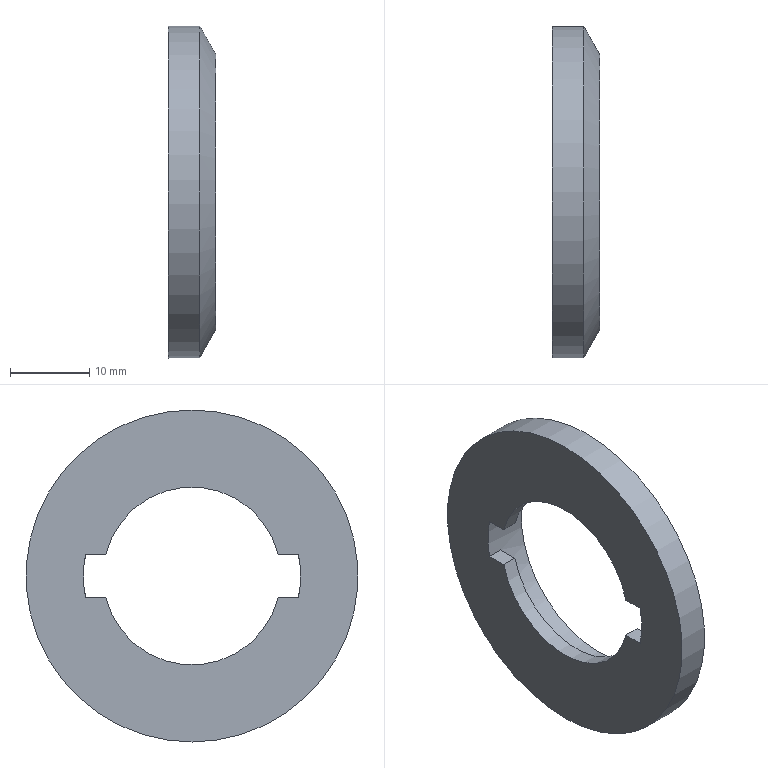Component | NX | SPACER_BLOCK | 1 solid | 13 faces | box 6 x 42 x 42 mm | volume 4639 mm3 | plane 8 | cylinder 4 | cone 1 | commonest cylinder face diameters 22.5 x2 42 x1 27.5 x1
STEP:
#1=CARTESIAN_POINT('',(0.,0.,0.));
#2=DIRECTION('',(0.,0.,1.));
#3=DIRECTION('',(1.,0.,0.));
#4=AXIS2_PLACEMENT_3D('',#1,#2,#3);
#5=CARTESIAN_POINT('',(-2.738,-11.881,-14.373));
#6=VERTEX_POINT('',#5);
#7=CARTESIAN_POINT('',(-2.738,-9.319,-14.373));
#8=VERTEX_POINT('',#7);
#9=CARTESIAN_POINT('',(-2.738,-11.881,-14.373));
#10=DIRECTION('',(0.,1.,0.));
#11=VECTOR('',#10,1.);
#12=LINE('',#9,#11);
#13=CARTESIAN_POINT('',(-2.738,1.601,-11.667));
#14=DIRECTION('',(-1.,0.,0.));
#15=DIRECTION('',(0.,0.,1.));
#16=AXIS2_PLACEMENT_3D('',#13,#14,#15);
#17=PLANE('',#16);
#18=CARTESIAN_POINT('',(-2.706,-13.481));
#19=DIRECTION('',(0.,1.));
#20=VECTOR('',#19,1.);
#21=LINE('',#18,#20);
#22=(GEOMETRIC_REPRESENTATION_CONTEXT(2)PARAMETRIC_REPRESENTATION_CONTEXT()REPRESENTATION_CONTEXT('',''));
#23=DEFINITIONAL_REPRESENTATION('',(#21),#22);
#24=PCURVE('',#17,#23);
#25=CARTESIAN_POINT('',(-12.738,-11.881,-14.373));
#26=DIRECTION('',(0.,0.,-1.));
#27=DIRECTION('',(0.,1.,0.));
#28=AXIS2_PLACEMENT_3D('',#25,#26,#27);
#29=PLANE('',#28);
#30=CARTESIAN_POINT('',(0.,10.));
#31=DIRECTION('',(1.,0.));
#32=VECTOR('',#31,1.);
#33=LINE('',#30,#32);
#34=(GEOMETRIC_REPRESENTATION_CONTEXT(2)PARAMETRIC_REPRESENTATION_CONTEXT()REPRESENTATION_CONTEXT('',''));
#35=DEFINITIONAL_REPRESENTATION('',(#33),#34);
#36=PCURVE('',#29,#35);
#37=SURFACE_CURVE('',#12,(#24,#36),.PCURVE_S1.);
#38=EDGE_CURVE('',#6,#8,#37,.T.);
#39=ORIENTED_EDGE('',*,*,#38,.F.);
#40=CARTESIAN_POINT('',(-2.738,1.601,-25.417));
#41=VERTEX_POINT('',#40);
#42=CARTESIAN_POINT('',(-2.738,1.601,-11.667));
#43=DIRECTION('',(-1.,0.,0.));
#44=DIRECTION('',(0.,0.,-1.));
#45=AXIS2_PLACEMENT_3D('',#42,#43,#44);
#46=CIRCLE('',#45,13.75);
#47=CARTESIAN_POINT('',(0.,0.));
#48=DIRECTION('',(-1.,0.));
#49=AXIS2_PLACEMENT_2D('',#47,#48);
#50=CIRCLE('',#49,13.75);
#51=(GEOMETRIC_REPRESENTATION_CONTEXT(2)PARAMETRIC_REPRESENTATION_CONTEXT()REPRESENTATION_CONTEXT('',''));
#52=DEFINITIONAL_REPRESENTATION('',(#50),#51);
#53=PCURVE('',#17,#52);
#54=CARTESIAN_POINT('',(1.262,1.601,-11.667));
#55=DIRECTION('',(-1.,0.,0.));
#56=DIRECTION('',(0.,0.,-1.));
#57=AXIS2_PLACEMENT_3D('',#54,#55,#56);
#58=CYLINDRICAL_SURFACE('',#57,13.75);
#59=CARTESIAN_POINT('',(-6.283,4.));
#60=DIRECTION('',(1.,0.));
#61=VECTOR('',#60,1.);
#62=LINE('',#59,#61);
#63=(GEOMETRIC_REPRESENTATION_CONTEXT(2)PARAMETRIC_REPRESENTATION_CONTEXT()REPRESENTATION_CONTEXT('',''));
#64=DEFINITIONAL_REPRESENTATION('',(#62),#63);
#65=PCURVE('',#58,#64);
#66=SURFACE_CURVE('',#46,(#53,#65),.PCURVE_S1.);
#67=EDGE_CURVE('',#41,#6,#66,.T.);
#68=ORIENTED_EDGE('',*,*,#67,.F.);
#69=CARTESIAN_POINT('',(-2.738,15.082,-14.373));
#70=VERTEX_POINT('',#69);
#71=CARTESIAN_POINT('',(-2.738,1.601,-11.667));
#72=DIRECTION('',(-1.,0.,0.));
#73=DIRECTION('',(0.,0.,-1.));
#74=AXIS2_PLACEMENT_3D('',#71,#72,#73);
#75=CIRCLE('',#74,13.75);
#76=CARTESIAN_POINT('',(0.,0.));
#77=DIRECTION('',(-1.,0.));
#78=AXIS2_PLACEMENT_2D('',#76,#77);
#79=CIRCLE('',#78,13.75);
#80=(GEOMETRIC_REPRESENTATION_CONTEXT(2)PARAMETRIC_REPRESENTATION_CONTEXT()REPRESENTATION_CONTEXT('',''));
#81=DEFINITIONAL_REPRESENTATION('',(#79),#80);
#82=PCURVE('',#17,#81);
#83=CARTESIAN_POINT('',(0.,4.));
#84=DIRECTION('',(1.,0.));
#85=VECTOR('',#84,1.);
#86=LINE('',#83,#85);
#87=(GEOMETRIC_REPRESENTATION_CONTEXT(2)PARAMETRIC_REPRESENTATION_CONTEXT()REPRESENTATION_CONTEXT('',''));
#88=DEFINITIONAL_REPRESENTATION('',(#86),#87);
#89=PCURVE('',#58,#88);
#90=SURFACE_CURVE('',#75,(#82,#89),.PCURVE_S1.);
#91=EDGE_CURVE('',#70,#41,#90,.T.);
#92=ORIENTED_EDGE('',*,*,#91,.F.);
#93=CARTESIAN_POINT('',(-2.738,12.52,-14.373));
#94=VERTEX_POINT('',#93);
#95=CARTESIAN_POINT('',(-2.738,12.52,-14.373));
#96=DIRECTION('',(0.,1.,0.));
#97=VECTOR('',#96,1.);
#98=LINE('',#95,#97);
#99=CARTESIAN_POINT('',(-2.706,10.92));
#100=DIRECTION('',(0.,1.));
#101=VECTOR('',#100,1.);
#102=LINE('',#99,#101);
#103=(GEOMETRIC_REPRESENTATION_CONTEXT(2)PARAMETRIC_REPRESENTATION_CONTEXT()REPRESENTATION_CONTEXT('',''));
#104=DEFINITIONAL_REPRESENTATION('',(#102),#103);
#105=PCURVE('',#17,#104);
#106=CARTESIAN_POINT('',(-12.738,12.52,-14.373));
#107=DIRECTION('',(0.,0.,-1.));
#108=DIRECTION('',(0.,1.,0.));
#109=AXIS2_PLACEMENT_3D('',#106,#107,#108);
#110=PLANE('',#109);
#111=CARTESIAN_POINT('',(0.,10.));
#112=DIRECTION('',(1.,0.));
#113=VECTOR('',#112,1.);
#114=LINE('',#111,#113);
#115=(GEOMETRIC_REPRESENTATION_CONTEXT(2)PARAMETRIC_REPRESENTATION_CONTEXT()REPRESENTATION_CONTEXT('',''));
#116=DEFINITIONAL_REPRESENTATION('',(#114),#115);
#117=PCURVE('',#110,#116);
#118=SURFACE_CURVE('',#98,(#105,#117),.PCURVE_S1.);
#119=EDGE_CURVE('',#94,#70,#118,.T.);
#120=ORIENTED_EDGE('',*,*,#119,.F.);
#121=CARTESIAN_POINT('',(-2.738,1.601,-11.667));
#122=DIRECTION('',(1.,0.,0.));
#123=DIRECTION('',(0.,0.,-1.));
#124=AXIS2_PLACEMENT_3D('',#121,#122,#123);
#125=CIRCLE('',#124,11.25);
#126=CARTESIAN_POINT('',(-11.25,0.));
#127=CARTESIAN_POINT('',(-11.25,19.486));
#128=CARTESIAN_POINT('',(5.625,9.743));
#129=CARTESIAN_POINT('',(22.5,0.));
#130=CARTESIAN_POINT('',(5.625,-9.743));
#131=CARTESIAN_POINT('',(-11.25,-19.486));
#132=CARTESIAN_POINT('',(-11.25,0.));
#133=(BOUNDED_CURVE()B_SPLINE_CURVE(2,(#126,#127,#128,#129,#130,#131,#132),.UNSPECIFIED.,.T.,.F.)B_SPLINE_CURVE_WITH_KNOTS((1,2,2,2,2,1),(-2.094,0.,2.094,4.189,6.283,8.378),.UNSPECIFIED.)CURVE()GEOMETRIC_REPRESENTATION_ITEM()RATIONAL_B_SPLINE_CURVE((1.,0.5,1.,0.5,1.,0.5,1.))REPRESENTATION_ITEM(''));
#134=(GEOMETRIC_REPRESENTATION_CONTEXT(2)PARAMETRIC_REPRESENTATION_CONTEXT()REPRESENTATION_CONTEXT('',''));
#135=DEFINITIONAL_REPRESENTATION('',(#133),#134);
#136=PCURVE('',#17,#135);
#137=CARTESIAN_POINT('',(-12.738,1.601,-11.667));
#138=DIRECTION('',(1.,0.,0.));
#139=DIRECTION('',(0.,0.,-1.));
#140=AXIS2_PLACEMENT_3D('',#137,#138,#139);
#141=CYLINDRICAL_SURFACE('',#140,11.25);
#142=CARTESIAN_POINT('',(0.,10.));
#143=DIRECTION('',(1.,0.));
#144=VECTOR('',#143,1.);
#145=LINE('',#142,#144);
#146=(GEOMETRIC_REPRESENTATION_CONTEXT(2)PARAMETRIC_REPRESENTATION_CONTEXT()REPRESENTATION_CONTEXT('',''));
#147=DEFINITIONAL_REPRESENTATION('',(#145),#146);
#148=PCURVE('',#141,#147);
#149=SURFACE_CURVE('',#125,(#136,#148),.PCURVE_S1.);
#150=EDGE_CURVE('',#8,#94,#149,.T.);
#151=ORIENTED_EDGE('',*,*,#150,.F.);
#152=EDGE_LOOP('',(#39,#68,#92,#120,#151));
#153=FACE_BOUND('',#152,.T.);
#154=ADVANCED_FACE('',(#153),#17,.F.);
#155=CARTESIAN_POINT('',(-4.738,-11.881,-8.961));
#156=VERTEX_POINT('',#155);
#157=CARTESIAN_POINT('',(-4.738,-9.319,-8.961));
#158=VERTEX_POINT('',#157);
#159=CARTESIAN_POINT('',(-4.738,-19.399,-8.961));
#160=DIRECTION('',(0.,1.,0.));
#161=VECTOR('',#160,1.);
#162=LINE('',#159,#161);
#163=CARTESIAN_POINT('',(-4.738,-19.399,-11.667));
#164=DIRECTION('',(-1.,0.,0.));
#165=DIRECTION('',(0.,0.,1.));
#166=AXIS2_PLACEMENT_3D('',#163,#164,#165);
#167=PLANE('',#166);
#168=CARTESIAN_POINT('',(2.706,0.));
#169=DIRECTION('',(0.,1.));
#170=VECTOR('',#169,1.);
#171=LINE('',#168,#170);
#172=(GEOMETRIC_REPRESENTATION_CONTEXT(2)PARAMETRIC_REPRESENTATION_CONTEXT()REPRESENTATION_CONTEXT('',''));
#173=DEFINITIONAL_REPRESENTATION('',(#171),#172);
#174=PCURVE('',#167,#173);
#175=CARTESIAN_POINT('',(-12.738,-9.319,-8.961));
#176=DIRECTION('',(0.,-0.,1.));
#177=DIRECTION('',(0.,-1.,-0.));
#178=AXIS2_PLACEMENT_3D('',#175,#176,#177);
#179=PLANE('',#178);
#180=CARTESIAN_POINT('',(10.08,8.));
#181=DIRECTION('',(-1.,0.));
#182=VECTOR('',#181,1.);
#183=LINE('',#180,#182);
#184=(GEOMETRIC_REPRESENTATION_CONTEXT(2)PARAMETRIC_REPRESENTATION_CONTEXT()REPRESENTATION_CONTEXT('',''));
#185=DEFINITIONAL_REPRESENTATION('',(#183),#184);
#186=PCURVE('',#179,#185);
#187=SURFACE_CURVE('',#162,(#174,#186),.PCURVE_S1.);
#188=EDGE_CURVE('',#156,#158,#187,.T.);
#189=ORIENTED_EDGE('',*,*,#188,.F.);
#190=CARTESIAN_POINT('',(-4.738,-11.881,-14.373));
#191=VERTEX_POINT('',#190);
#192=CARTESIAN_POINT('',(-4.738,1.601,-11.667));
#193=DIRECTION('',(-1.,0.,0.));
#194=DIRECTION('',(0.,0.,1.));
#195=AXIS2_PLACEMENT_3D('',#192,#193,#194);
#196=CIRCLE('',#195,13.75);
#197=CARTESIAN_POINT('',(0.,21.));
#198=DIRECTION('',(1.,0.));
#199=AXIS2_PLACEMENT_2D('',#197,#198);
#200=CIRCLE('',#199,13.75);
#201=(GEOMETRIC_REPRESENTATION_CONTEXT(2)PARAMETRIC_REPRESENTATION_CONTEXT()REPRESENTATION_CONTEXT('',''));
#202=DEFINITIONAL_REPRESENTATION('',(#200),#201);
#203=PCURVE('',#167,#202);
#204=CARTESIAN_POINT('',(-3.142,6.));
#205=DIRECTION('',(1.,0.));
#206=VECTOR('',#205,1.);
#207=LINE('',#204,#206);
#208=(GEOMETRIC_REPRESENTATION_CONTEXT(2)PARAMETRIC_REPRESENTATION_CONTEXT()REPRESENTATION_CONTEXT('',''));
#209=DEFINITIONAL_REPRESENTATION('',(#207),#208);
#210=PCURVE('',#58,#209);
#211=SURFACE_CURVE('',#196,(#203,#210),.PCURVE_S1.);
#212=EDGE_CURVE('',#191,#156,#211,.T.);
#213=ORIENTED_EDGE('',*,*,#212,.F.);
#214=CARTESIAN_POINT('',(-4.738,-9.319,-14.373));
#215=VERTEX_POINT('',#214);
#216=CARTESIAN_POINT('',(-4.738,-19.399,-14.373));
#217=DIRECTION('',(0.,-1.,-0.));
#218=VECTOR('',#217,1.);
#219=LINE('',#216,#218);
#220=CARTESIAN_POINT('',(-2.706,0.));
#221=DIRECTION('',(-0.,-1.));
#222=VECTOR('',#221,1.);
#223=LINE('',#220,#222);
#224=(GEOMETRIC_REPRESENTATION_CONTEXT(2)PARAMETRIC_REPRESENTATION_CONTEXT()REPRESENTATION_CONTEXT('',''));
#225=DEFINITIONAL_REPRESENTATION('',(#223),#224);
#226=PCURVE('',#167,#225);
#227=CARTESIAN_POINT('',(-7.519,8.));
#228=DIRECTION('',(-1.,0.));
#229=VECTOR('',#228,1.);
#230=LINE('',#227,#229);
#231=(GEOMETRIC_REPRESENTATION_CONTEXT(2)PARAMETRIC_REPRESENTATION_CONTEXT()REPRESENTATION_CONTEXT('',''));
#232=DEFINITIONAL_REPRESENTATION('',(#230),#231);
#233=PCURVE('',#29,#232);
#234=SURFACE_CURVE('',#219,(#226,#233),.PCURVE_S1.);
#235=EDGE_CURVE('',#215,#191,#234,.T.);
#236=ORIENTED_EDGE('',*,*,#235,.F.);
#237=CARTESIAN_POINT('',(-4.738,12.52,-14.373));
#238=VERTEX_POINT('',#237);
#239=CARTESIAN_POINT('',(-4.738,1.601,-11.667));
#240=DIRECTION('',(-1.,0.,0.));
#241=DIRECTION('',(0.,0.,1.));
#242=AXIS2_PLACEMENT_3D('',#239,#240,#241);
#243=CIRCLE('',#242,11.25);
#244=CARTESIAN_POINT('',(0.,21.));
#245=DIRECTION('',(1.,0.));
#246=AXIS2_PLACEMENT_2D('',#244,#245);
#247=CIRCLE('',#246,11.25);
#248=(GEOMETRIC_REPRESENTATION_CONTEXT(2)PARAMETRIC_REPRESENTATION_CONTEXT()REPRESENTATION_CONTEXT('',''));
#249=DEFINITIONAL_REPRESENTATION('',(#247),#248);
#250=PCURVE('',#167,#249);
#251=CARTESIAN_POINT('',(9.425,8.));
#252=DIRECTION('',(-1.,0.));
#253=VECTOR('',#252,1.);
#254=LINE('',#251,#253);
#255=(GEOMETRIC_REPRESENTATION_CONTEXT(2)PARAMETRIC_REPRESENTATION_CONTEXT()REPRESENTATION_CONTEXT('',''));
#256=DEFINITIONAL_REPRESENTATION('',(#254),#255);
#257=PCURVE('',#141,#256);
#258=SURFACE_CURVE('',#243,(#250,#257),.PCURVE_S1.);
#259=EDGE_CURVE('',#238,#215,#258,.T.);
#260=ORIENTED_EDGE('',*,*,#259,.F.);
#261=CARTESIAN_POINT('',(-4.738,15.082,-14.373));
#262=VERTEX_POINT('',#261);
#263=CARTESIAN_POINT('',(-4.738,-19.399,-14.373));
#264=DIRECTION('',(0.,-1.,-0.));
#265=VECTOR('',#264,1.);
#266=LINE('',#263,#265);
#267=CARTESIAN_POINT('',(-2.706,0.));
#268=DIRECTION('',(-0.,-1.));
#269=VECTOR('',#268,1.);
#270=LINE('',#267,#269);
#271=(GEOMETRIC_REPRESENTATION_CONTEXT(2)PARAMETRIC_REPRESENTATION_CONTEXT()REPRESENTATION_CONTEXT('',''));
#272=DEFINITIONAL_REPRESENTATION('',(#270),#271);
#273=PCURVE('',#167,#272);
#274=CARTESIAN_POINT('',(-31.92,8.));
#275=DIRECTION('',(-1.,0.));
#276=VECTOR('',#275,1.);
#277=LINE('',#274,#276);
#278=(GEOMETRIC_REPRESENTATION_CONTEXT(2)PARAMETRIC_REPRESENTATION_CONTEXT()REPRESENTATION_CONTEXT('',''));
#279=DEFINITIONAL_REPRESENTATION('',(#277),#278);
#280=PCURVE('',#110,#279);
#281=SURFACE_CURVE('',#266,(#273,#280),.PCURVE_S1.);
#282=EDGE_CURVE('',#262,#238,#281,.T.);
#283=ORIENTED_EDGE('',*,*,#282,.F.);
#284=CARTESIAN_POINT('',(-4.738,15.082,-8.961));
#285=VERTEX_POINT('',#284);
#286=CARTESIAN_POINT('',(-4.738,1.601,-11.667));
#287=DIRECTION('',(-1.,0.,0.));
#288=DIRECTION('',(0.,0.,1.));
#289=AXIS2_PLACEMENT_3D('',#286,#287,#288);
#290=CIRCLE('',#289,13.75);
#291=CARTESIAN_POINT('',(0.,21.));
#292=DIRECTION('',(1.,0.));
#293=AXIS2_PLACEMENT_2D('',#291,#292);
#294=CIRCLE('',#293,13.75);
#295=(GEOMETRIC_REPRESENTATION_CONTEXT(2)PARAMETRIC_REPRESENTATION_CONTEXT()REPRESENTATION_CONTEXT('',''));
#296=DEFINITIONAL_REPRESENTATION('',(#294),#295);
#297=PCURVE('',#167,#296);
#298=CARTESIAN_POINT('',(3.142,6.));
#299=DIRECTION('',(1.,0.));
#300=VECTOR('',#299,1.);
#301=LINE('',#298,#300);
#302=(GEOMETRIC_REPRESENTATION_CONTEXT(2)PARAMETRIC_REPRESENTATION_CONTEXT()REPRESENTATION_CONTEXT('',''));
#303=DEFINITIONAL_REPRESENTATION('',(#301),#302);
#304=PCURVE('',#58,#303);
#305=SURFACE_CURVE('',#290,(#297,#304),.PCURVE_S1.);
#306=EDGE_CURVE('',#285,#262,#305,.T.);
#307=ORIENTED_EDGE('',*,*,#306,.F.);
#308=CARTESIAN_POINT('',(-4.738,12.52,-8.961));
#309=VERTEX_POINT('',#308);
#310=CARTESIAN_POINT('',(-4.738,-19.399,-8.961));
#311=DIRECTION('',(0.,1.,0.));
#312=VECTOR('',#311,1.);
#313=LINE('',#310,#312);
#314=CARTESIAN_POINT('',(2.706,0.));
#315=DIRECTION('',(0.,1.));
#316=VECTOR('',#315,1.);
#317=LINE('',#314,#316);
#318=(GEOMETRIC_REPRESENTATION_CONTEXT(2)PARAMETRIC_REPRESENTATION_CONTEXT()REPRESENTATION_CONTEXT('',''));
#319=DEFINITIONAL_REPRESENTATION('',(#317),#318);
#320=PCURVE('',#167,#319);
#321=CARTESIAN_POINT('',(-12.738,15.082,-8.961));
#322=DIRECTION('',(0.,-0.,1.));
#323=DIRECTION('',(0.,-1.,-0.));
#324=AXIS2_PLACEMENT_3D('',#321,#322,#323);
#325=PLANE('',#324);
#326=CARTESIAN_POINT('',(34.481,8.));
#327=DIRECTION('',(-1.,0.));
#328=VECTOR('',#327,1.);
#329=LINE('',#326,#328);
#330=(GEOMETRIC_REPRESENTATION_CONTEXT(2)PARAMETRIC_REPRESENTATION_CONTEXT()REPRESENTATION_CONTEXT('',''));
#331=DEFINITIONAL_REPRESENTATION('',(#329),#330);
#332=PCURVE('',#325,#331);
#333=SURFACE_CURVE('',#313,(#320,#332),.PCURVE_S1.);
#334=EDGE_CURVE('',#309,#285,#333,.T.);
#335=ORIENTED_EDGE('',*,*,#334,.F.);
#336=CARTESIAN_POINT('',(-4.738,1.601,-11.667));
#337=DIRECTION('',(-1.,0.,0.));
#338=DIRECTION('',(0.,0.,1.));
#339=AXIS2_PLACEMENT_3D('',#336,#337,#338);
#340=CIRCLE('',#339,11.25);
#341=CARTESIAN_POINT('',(0.,21.));
#342=DIRECTION('',(1.,0.));
#343=AXIS2_PLACEMENT_2D('',#341,#342);
#344=CIRCLE('',#343,11.25);
#345=(GEOMETRIC_REPRESENTATION_CONTEXT(2)PARAMETRIC_REPRESENTATION_CONTEXT()REPRESENTATION_CONTEXT('',''));
#346=DEFINITIONAL_REPRESENTATION('',(#344),#345);
#347=PCURVE('',#167,#346);
#348=CARTESIAN_POINT('',(-12.738,1.601,-11.667));
#349=DIRECTION('',(1.,0.,0.));
#350=DIRECTION('',(0.,0.,-1.));
#351=AXIS2_PLACEMENT_3D('',#348,#349,#350);
#352=CYLINDRICAL_SURFACE('',#351,11.25);
#353=CARTESIAN_POINT('',(9.425,8.));
#354=DIRECTION('',(-1.,0.));
#355=VECTOR('',#354,1.);
#356=LINE('',#353,#355);
#357=(GEOMETRIC_REPRESENTATION_CONTEXT(2)PARAMETRIC_REPRESENTATION_CONTEXT()REPRESENTATION_CONTEXT('',''));
#358=DEFINITIONAL_REPRESENTATION('',(#356),#357);
#359=PCURVE('',#352,#358);
#360=SURFACE_CURVE('',#340,(#347,#359),.PCURVE_S1.);
#361=EDGE_CURVE('',#158,#309,#360,.T.);
#362=ORIENTED_EDGE('',*,*,#361,.F.);
#363=EDGE_LOOP('',(#189,#213,#236,#260,#283,#307,#335,#362));
#364=FACE_BOUND('',#363,.T.);
#365=CARTESIAN_POINT('',(-4.738,1.601,-32.667));
#366=VERTEX_POINT('',#365);
#367=CARTESIAN_POINT('',(-4.738,1.601,-11.667));
#368=DIRECTION('',(1.,0.,0.));
#369=DIRECTION('',(0.,0.,-1.));
#370=AXIS2_PLACEMENT_3D('',#367,#368,#369);
#371=CIRCLE('',#370,21.);
#372=CARTESIAN_POINT('',(-21.,21.));
#373=CARTESIAN_POINT('',(-21.,57.373));
#374=CARTESIAN_POINT('',(10.5,39.187));
#375=CARTESIAN_POINT('',(42.,21.));
#376=CARTESIAN_POINT('',(10.5,2.813));
#377=CARTESIAN_POINT('',(-21.,-15.373));
#378=CARTESIAN_POINT('',(-21.,21.));
#379=(BOUNDED_CURVE()B_SPLINE_CURVE(2,(#372,#373,#374,#375,#376,#377,#378),.UNSPECIFIED.,.T.,.F.)B_SPLINE_CURVE_WITH_KNOTS((1,2,2,2,2,1),(-2.094,0.,2.094,4.189,6.283,8.378),.UNSPECIFIED.)CURVE()GEOMETRIC_REPRESENTATION_ITEM()RATIONAL_B_SPLINE_CURVE((1.,0.5,1.,0.5,1.,0.5,1.))REPRESENTATION_ITEM(''));
#380=(GEOMETRIC_REPRESENTATION_CONTEXT(2)PARAMETRIC_REPRESENTATION_CONTEXT()REPRESENTATION_CONTEXT('',''));
#381=DEFINITIONAL_REPRESENTATION('',(#379),#380);
#382=PCURVE('',#167,#381);
#383=CARTESIAN_POINT('',(-4.738,1.601,-11.667));
#384=DIRECTION('',(1.,0.,0.));
#385=DIRECTION('',(0.,0.,-1.));
#386=AXIS2_PLACEMENT_3D('',#383,#384,#385);
#387=CYLINDRICAL_SURFACE('',#386,21.);
#388=CARTESIAN_POINT('',(0.,0.));
#389=DIRECTION('',(1.,0.));
#390=VECTOR('',#389,1.);
#391=LINE('',#388,#390);
#392=(GEOMETRIC_REPRESENTATION_CONTEXT(2)PARAMETRIC_REPRESENTATION_CONTEXT()REPRESENTATION_CONTEXT('',''));
#393=DEFINITIONAL_REPRESENTATION('',(#391),#392);
#394=PCURVE('',#387,#393);
#395=SURFACE_CURVE('',#371,(#382,#394),.PCURVE_S1.);
#396=EDGE_CURVE('',#366,#366,#395,.T.);
#397=ORIENTED_EDGE('',*,*,#396,.F.);
#398=EDGE_LOOP('',(#397));
#399=FACE_BOUND('',#398,.T.);
#400=ADVANCED_FACE('',(#364,#399),#167,.T.);
#401=ORIENTED_EDGE('',*,*,#396,.T.);
#402=CARTESIAN_POINT('',(-0.7381,1.601,-32.667));
#403=VERTEX_POINT('',#402);
#404=CARTESIAN_POINT('',(-4.738,1.601,-32.667));
#405=CARTESIAN_POINT('',(-0.7381,1.601,-32.667));
#406=B_SPLINE_CURVE_WITH_KNOTS('',1,(#404,#405),.UNSPECIFIED.,.F.,.F.,(2,2),(0.,4.),.PIECEWISE_BEZIER_KNOTS.);
#407=CARTESIAN_POINT('',(6.283,0.));
#408=DIRECTION('',(0.,1.));
#409=VECTOR('',#408,1.);
#410=LINE('',#407,#409);
#411=(GEOMETRIC_REPRESENTATION_CONTEXT(2)PARAMETRIC_REPRESENTATION_CONTEXT()REPRESENTATION_CONTEXT('',''));
#412=DEFINITIONAL_REPRESENTATION('',(#410),#411);
#413=PCURVE('',#387,#412);
#414=CARTESIAN_POINT('',(0.,0.));
#415=DIRECTION('',(0.,1.));
#416=VECTOR('',#415,1.);
#417=LINE('',#414,#416);
#418=(GEOMETRIC_REPRESENTATION_CONTEXT(2)PARAMETRIC_REPRESENTATION_CONTEXT()REPRESENTATION_CONTEXT('',''));
#419=DEFINITIONAL_REPRESENTATION('',(#417),#418);
#420=PCURVE('',#387,#419);
#421=SEAM_CURVE('',#406,(#413,#420),.PCURVE_S1.);
#422=EDGE_CURVE('',#366,#403,#421,.T.);
#423=ORIENTED_EDGE('',*,*,#422,.T.);
#424=CARTESIAN_POINT('',(-0.7381,1.601,-11.667));
#425=DIRECTION('',(1.,0.,0.));
#426=DIRECTION('',(0.,0.,-1.));
#427=AXIS2_PLACEMENT_3D('',#424,#425,#426);
#428=CIRCLE('',#427,21.);
#429=CARTESIAN_POINT('',(0.,4.));
#430=DIRECTION('',(1.,0.));
#431=VECTOR('',#430,1.);
#432=LINE('',#429,#431);
#433=(GEOMETRIC_REPRESENTATION_CONTEXT(2)PARAMETRIC_REPRESENTATION_CONTEXT()REPRESENTATION_CONTEXT('',''));
#434=DEFINITIONAL_REPRESENTATION('',(#432),#433);
#435=PCURVE('',#387,#434);
#436=CARTESIAN_POINT('',(1.262,1.601,-11.667));
#437=DIRECTION('',(-1.,0.,0.));
#438=DIRECTION('',(0.,0.,1.));
#439=AXIS2_PLACEMENT_3D('',#436,#437,#438);
#440=CONICAL_SURFACE('',#439,17.4,1.064);
#441=CARTESIAN_POINT('',(9.425,2.));
#442=DIRECTION('',(-1.,0.));
#443=VECTOR('',#442,1.);
#444=LINE('',#441,#443);
#445=(GEOMETRIC_REPRESENTATION_CONTEXT(2)PARAMETRIC_REPRESENTATION_CONTEXT()REPRESENTATION_CONTEXT('',''));
#446=DEFINITIONAL_REPRESENTATION('',(#444),#445);
#447=PCURVE('',#440,#446);
#448=SURFACE_CURVE('',#428,(#435,#447),.PCURVE_S1.);
#449=EDGE_CURVE('',#403,#403,#448,.T.);
#450=ORIENTED_EDGE('',*,*,#449,.F.);
#451=ORIENTED_EDGE('',*,*,#422,.F.);
#452=EDGE_LOOP('',(#401,#423,#450,#451));
#453=FACE_BOUND('',#452,.T.);
#454=ADVANCED_FACE('',(#453),#387,.T.);
#455=ORIENTED_EDGE('',*,*,#449,.T.);
#456=CARTESIAN_POINT('',(1.262,1.601,-29.067));
#457=VERTEX_POINT('',#456);
#458=CARTESIAN_POINT('',(1.262,1.601,-29.067));
#459=CARTESIAN_POINT('',(-0.7381,1.601,-32.667));
#460=B_SPLINE_CURVE_WITH_KNOTS('',1,(#458,#459),.UNSPECIFIED.,.F.,.F.,(2,2),(0.,4.118),.PIECEWISE_BEZIER_KNOTS.);
#461=CARTESIAN_POINT('',(3.142,0.));
#462=DIRECTION('',(0.,1.));
#463=VECTOR('',#462,1.);
#464=LINE('',#461,#463);
#465=(GEOMETRIC_REPRESENTATION_CONTEXT(2)PARAMETRIC_REPRESENTATION_CONTEXT()REPRESENTATION_CONTEXT('',''));
#466=DEFINITIONAL_REPRESENTATION('',(#464),#465);
#467=PCURVE('',#440,#466);
#468=CARTESIAN_POINT('',(9.425,0.));
#469=DIRECTION('',(0.,1.));
#470=VECTOR('',#469,1.);
#471=LINE('',#468,#470);
#472=(GEOMETRIC_REPRESENTATION_CONTEXT(2)PARAMETRIC_REPRESENTATION_CONTEXT()REPRESENTATION_CONTEXT('',''));
#473=DEFINITIONAL_REPRESENTATION('',(#471),#472);
#474=PCURVE('',#440,#473);
#475=SEAM_CURVE('',#460,(#467,#474),.PCURVE_S1.);
#476=EDGE_CURVE('',#457,#403,#475,.T.);
#477=ORIENTED_EDGE('',*,*,#476,.F.);
#478=CARTESIAN_POINT('',(1.262,1.601,-11.667));
#479=DIRECTION('',(1.,0.,0.));
#480=DIRECTION('',(0.,0.,-1.));
#481=AXIS2_PLACEMENT_3D('',#478,#479,#480);
#482=CIRCLE('',#481,17.4);
#483=CARTESIAN_POINT('',(9.425,0.));
#484=DIRECTION('',(-1.,0.));
#485=VECTOR('',#484,1.);
#486=LINE('',#483,#485);
#487=(GEOMETRIC_REPRESENTATION_CONTEXT(2)PARAMETRIC_REPRESENTATION_CONTEXT()REPRESENTATION_CONTEXT('',''));
#488=DEFINITIONAL_REPRESENTATION('',(#486),#487);
#489=PCURVE('',#440,#488);
#490=CARTESIAN_POINT('',(1.262,1.601,-11.667));
#491=DIRECTION('',(1.,0.,0.));
#492=DIRECTION('',(0.,0.,-1.));
#493=AXIS2_PLACEMENT_3D('',#490,#491,#492);
#494=PLANE('',#493);
#495=CARTESIAN_POINT('',(0.,0.));
#496=DIRECTION('',(1.,0.));
#497=AXIS2_PLACEMENT_2D('',#495,#496);
#498=CIRCLE('',#497,17.4);
#499=(GEOMETRIC_REPRESENTATION_CONTEXT(2)PARAMETRIC_REPRESENTATION_CONTEXT()REPRESENTATION_CONTEXT('',''));
#500=DEFINITIONAL_REPRESENTATION('',(#498),#499);
#501=PCURVE('',#494,#500);
#502=SURFACE_CURVE('',#482,(#489,#501),.PCURVE_S1.);
#503=EDGE_CURVE('',#457,#457,#502,.T.);
#504=ORIENTED_EDGE('',*,*,#503,.F.);
#505=ORIENTED_EDGE('',*,*,#476,.T.);
#506=EDGE_LOOP('',(#455,#477,#504,#505));
#507=FACE_BOUND('',#506,.T.);
#508=ADVANCED_FACE('',(#507),#440,.T.);
#509=CARTESIAN_POINT('',(1.262,1.601,-25.417));
#510=VERTEX_POINT('',#509);
#511=CARTESIAN_POINT('',(1.262,1.601,-11.667));
#512=DIRECTION('',(-1.,0.,0.));
#513=DIRECTION('',(0.,0.,-1.));
#514=AXIS2_PLACEMENT_3D('',#511,#512,#513);
#515=CIRCLE('',#514,13.75);
#516=CARTESIAN_POINT('',(13.75,0.));
#517=CARTESIAN_POINT('',(13.75,-23.816));
#518=CARTESIAN_POINT('',(-6.875,-11.908));
#519=CARTESIAN_POINT('',(-27.5,-0.));
#520=CARTESIAN_POINT('',(-6.875,11.908));
#521=CARTESIAN_POINT('',(13.75,23.816));
#522=CARTESIAN_POINT('',(13.75,0.));
#523=(BOUNDED_CURVE()B_SPLINE_CURVE(2,(#516,#517,#518,#519,#520,#521,#522),.UNSPECIFIED.,.T.,.F.)B_SPLINE_CURVE_WITH_KNOTS((1,2,2,2,2,1),(-2.094,0.,2.094,4.189,6.283,8.378),.UNSPECIFIED.)CURVE()GEOMETRIC_REPRESENTATION_ITEM()RATIONAL_B_SPLINE_CURVE((1.,0.5,1.,0.5,1.,0.5,1.))REPRESENTATION_ITEM(''));
#524=(GEOMETRIC_REPRESENTATION_CONTEXT(2)PARAMETRIC_REPRESENTATION_CONTEXT()REPRESENTATION_CONTEXT('',''));
#525=DEFINITIONAL_REPRESENTATION('',(#523),#524);
#526=PCURVE('',#494,#525);
#527=CARTESIAN_POINT('',(0.,0.));
#528=DIRECTION('',(1.,0.));
#529=VECTOR('',#528,1.);
#530=LINE('',#527,#529);
#531=(GEOMETRIC_REPRESENTATION_CONTEXT(2)PARAMETRIC_REPRESENTATION_CONTEXT()REPRESENTATION_CONTEXT('',''));
#532=DEFINITIONAL_REPRESENTATION('',(#530),#531);
#533=PCURVE('',#58,#532);
#534=SURFACE_CURVE('',#515,(#526,#533),.PCURVE_S1.);
#535=EDGE_CURVE('',#510,#510,#534,.T.);
#536=ORIENTED_EDGE('',*,*,#535,.T.);
#537=EDGE_LOOP('',(#536));
#538=FACE_BOUND('',#537,.T.);
#539=ORIENTED_EDGE('',*,*,#503,.T.);
#540=EDGE_LOOP('',(#539));
#541=FACE_BOUND('',#540,.T.);
#542=ADVANCED_FACE('',(#538,#541),#494,.T.);
#543=CARTESIAN_POINT('',(-2.738,-9.319,-8.961));
#544=VERTEX_POINT('',#543);
#545=CARTESIAN_POINT('',(-2.738,-11.881,-8.961));
#546=VERTEX_POINT('',#545);
#547=CARTESIAN_POINT('',(-2.738,-9.319,-8.961));
#548=DIRECTION('',(0.,-1.,-0.));
#549=VECTOR('',#548,1.);
#550=LINE('',#547,#549);
#551=CARTESIAN_POINT('',(-2.738,1.601,-11.667));
#552=DIRECTION('',(-1.,0.,0.));
#553=DIRECTION('',(0.,0.,1.));
#554=AXIS2_PLACEMENT_3D('',#551,#552,#553);
#555=PLANE('',#554);
#556=CARTESIAN_POINT('',(2.706,-10.92));
#557=DIRECTION('',(-0.,-1.));
#558=VECTOR('',#557,1.);
#559=LINE('',#556,#558);
#560=(GEOMETRIC_REPRESENTATION_CONTEXT(2)PARAMETRIC_REPRESENTATION_CONTEXT()REPRESENTATION_CONTEXT('',''));
#561=DEFINITIONAL_REPRESENTATION('',(#559),#560);
#562=PCURVE('',#555,#561);
#563=CARTESIAN_POINT('',(0.,10.));
#564=DIRECTION('',(1.,0.));
#565=VECTOR('',#564,1.);
#566=LINE('',#563,#565);
#567=(GEOMETRIC_REPRESENTATION_CONTEXT(2)PARAMETRIC_REPRESENTATION_CONTEXT()REPRESENTATION_CONTEXT('',''));
#568=DEFINITIONAL_REPRESENTATION('',(#566),#567);
#569=PCURVE('',#179,#568);
#570=SURFACE_CURVE('',#550,(#562,#569),.PCURVE_S1.);
#571=EDGE_CURVE('',#544,#546,#570,.T.);
#572=ORIENTED_EDGE('',*,*,#571,.F.);
#573=CARTESIAN_POINT('',(-2.738,12.52,-8.961));
#574=VERTEX_POINT('',#573);
#575=CARTESIAN_POINT('',(-2.738,1.601,-11.667));
#576=DIRECTION('',(1.,0.,0.));
#577=DIRECTION('',(0.,0.,-1.));
#578=AXIS2_PLACEMENT_3D('',#575,#576,#577);
#579=CIRCLE('',#578,11.25);
#580=CARTESIAN_POINT('',(-11.25,0.));
#581=CARTESIAN_POINT('',(-11.25,19.486));
#582=CARTESIAN_POINT('',(5.625,9.743));
#583=CARTESIAN_POINT('',(22.5,0.));
#584=CARTESIAN_POINT('',(5.625,-9.743));
#585=CARTESIAN_POINT('',(-11.25,-19.486));
#586=CARTESIAN_POINT('',(-11.25,0.));
#587=(BOUNDED_CURVE()B_SPLINE_CURVE(2,(#580,#581,#582,#583,#584,#585,#586),.UNSPECIFIED.,.T.,.F.)B_SPLINE_CURVE_WITH_KNOTS((1,2,2,2,2,1),(-2.094,0.,2.094,4.189,6.283,8.378),.UNSPECIFIED.)CURVE()GEOMETRIC_REPRESENTATION_ITEM()RATIONAL_B_SPLINE_CURVE((1.,0.5,1.,0.5,1.,0.5,1.))REPRESENTATION_ITEM(''));
#588=(GEOMETRIC_REPRESENTATION_CONTEXT(2)PARAMETRIC_REPRESENTATION_CONTEXT()REPRESENTATION_CONTEXT('',''));
#589=DEFINITIONAL_REPRESENTATION('',(#587),#588);
#590=PCURVE('',#555,#589);
#591=CARTESIAN_POINT('',(0.,10.));
#592=DIRECTION('',(1.,0.));
#593=VECTOR('',#592,1.);
#594=LINE('',#591,#593);
#595=(GEOMETRIC_REPRESENTATION_CONTEXT(2)PARAMETRIC_REPRESENTATION_CONTEXT()REPRESENTATION_CONTEXT('',''));
#596=DEFINITIONAL_REPRESENTATION('',(#594),#595);
#597=PCURVE('',#352,#596);
#598=SURFACE_CURVE('',#579,(#590,#597),.PCURVE_S1.);
#599=EDGE_CURVE('',#574,#544,#598,.T.);
#600=ORIENTED_EDGE('',*,*,#599,.F.);
#601=CARTESIAN_POINT('',(-2.738,15.082,-8.961));
#602=VERTEX_POINT('',#601);
#603=CARTESIAN_POINT('',(-2.738,15.082,-8.961));
#604=DIRECTION('',(0.,-1.,-0.));
#605=VECTOR('',#604,1.);
#606=LINE('',#603,#605);
#607=CARTESIAN_POINT('',(2.706,13.481));
#608=DIRECTION('',(-0.,-1.));
#609=VECTOR('',#608,1.);
#610=LINE('',#607,#609);
#611=(GEOMETRIC_REPRESENTATION_CONTEXT(2)PARAMETRIC_REPRESENTATION_CONTEXT()REPRESENTATION_CONTEXT('',''));
#612=DEFINITIONAL_REPRESENTATION('',(#610),#611);
#613=PCURVE('',#555,#612);
#614=CARTESIAN_POINT('',(0.,10.));
#615=DIRECTION('',(1.,0.));
#616=VECTOR('',#615,1.);
#617=LINE('',#614,#616);
#618=(GEOMETRIC_REPRESENTATION_CONTEXT(2)PARAMETRIC_REPRESENTATION_CONTEXT()REPRESENTATION_CONTEXT('',''));
#619=DEFINITIONAL_REPRESENTATION('',(#617),#618);
#620=PCURVE('',#325,#619);
#621=SURFACE_CURVE('',#606,(#613,#620),.PCURVE_S1.);
#622=EDGE_CURVE('',#602,#574,#621,.T.);
#623=ORIENTED_EDGE('',*,*,#622,.F.);
#624=CARTESIAN_POINT('',(-2.738,1.601,-11.667));
#625=DIRECTION('',(-1.,0.,0.));
#626=DIRECTION('',(0.,0.,-1.));
#627=AXIS2_PLACEMENT_3D('',#624,#625,#626);
#628=CIRCLE('',#627,13.75);
#629=CARTESIAN_POINT('',(0.,0.));
#630=DIRECTION('',(-1.,0.));
#631=AXIS2_PLACEMENT_2D('',#629,#630);
#632=CIRCLE('',#631,13.75);
#633=(GEOMETRIC_REPRESENTATION_CONTEXT(2)PARAMETRIC_REPRESENTATION_CONTEXT()REPRESENTATION_CONTEXT('',''));
#634=DEFINITIONAL_REPRESENTATION('',(#632),#633);
#635=PCURVE('',#555,#634);
#636=CARTESIAN_POINT('',(0.,4.));
#637=DIRECTION('',(1.,0.));
#638=VECTOR('',#637,1.);
#639=LINE('',#636,#638);
#640=(GEOMETRIC_REPRESENTATION_CONTEXT(2)PARAMETRIC_REPRESENTATION_CONTEXT()REPRESENTATION_CONTEXT('',''));
#641=DEFINITIONAL_REPRESENTATION('',(#639),#640);
#642=PCURVE('',#58,#641);
#643=SURFACE_CURVE('',#628,(#635,#642),.PCURVE_S1.);
#644=EDGE_CURVE('',#546,#602,#643,.T.);
#645=ORIENTED_EDGE('',*,*,#644,.F.);
#646=EDGE_LOOP('',(#572,#600,#623,#645));
#647=FACE_BOUND('',#646,.T.);
#648=ADVANCED_FACE('',(#647),#555,.F.);
#649=CARTESIAN_POINT('',(-12.738,15.082,-14.373));
#650=DIRECTION('',(1.,0.,0.));
#651=VECTOR('',#650,1.);
#652=LINE('',#649,#651);
#653=CARTESIAN_POINT('',(4.91,14.));
#654=DIRECTION('',(0.,-1.));
#655=VECTOR('',#654,1.);
#656=LINE('',#653,#655);
#657=(GEOMETRIC_REPRESENTATION_CONTEXT(2)PARAMETRIC_REPRESENTATION_CONTEXT()REPRESENTATION_CONTEXT('',''));
#658=DEFINITIONAL_REPRESENTATION('',(#656),#657);
#659=PCURVE('',#58,#658);
#660=CARTESIAN_POINT('',(2.561,0.));
#661=DIRECTION('',(0.,1.));
#662=VECTOR('',#661,1.);
#663=LINE('',#660,#662);
#664=(GEOMETRIC_REPRESENTATION_CONTEXT(2)PARAMETRIC_REPRESENTATION_CONTEXT()REPRESENTATION_CONTEXT('',''));
#665=DEFINITIONAL_REPRESENTATION('',(#663),#664);
#666=PCURVE('',#110,#665);
#667=SURFACE_CURVE('',#652,(#659,#666),.PCURVE_S1.);
#668=EDGE_CURVE('',#262,#70,#667,.T.);
#669=ORIENTED_EDGE('',*,*,#668,.F.);
#670=ORIENTED_EDGE('',*,*,#306,.F.);
#671=CARTESIAN_POINT('',(-12.738,15.082,-8.961));
#672=DIRECTION('',(1.,0.,0.));
#673=VECTOR('',#672,1.);
#674=LINE('',#671,#673);
#675=CARTESIAN_POINT('',(4.514,14.));
#676=DIRECTION('',(0.,-1.));
#677=VECTOR('',#676,1.);
#678=LINE('',#675,#677);
#679=(GEOMETRIC_REPRESENTATION_CONTEXT(2)PARAMETRIC_REPRESENTATION_CONTEXT()REPRESENTATION_CONTEXT('',''));
#680=DEFINITIONAL_REPRESENTATION('',(#678),#679);
#681=PCURVE('',#58,#680);
#682=CARTESIAN_POINT('',(0.,0.));
#683=DIRECTION('',(0.,1.));
#684=VECTOR('',#683,1.);
#685=LINE('',#682,#684);
#686=(GEOMETRIC_REPRESENTATION_CONTEXT(2)PARAMETRIC_REPRESENTATION_CONTEXT()REPRESENTATION_CONTEXT('',''));
#687=DEFINITIONAL_REPRESENTATION('',(#685),#686);
#688=PCURVE('',#325,#687);
#689=SURFACE_CURVE('',#674,(#681,#688),.PCURVE_S1.);
#690=EDGE_CURVE('',#285,#602,#689,.T.);
#691=ORIENTED_EDGE('',*,*,#690,.T.);
#692=ORIENTED_EDGE('',*,*,#644,.F.);
#693=CARTESIAN_POINT('',(-12.738,-11.881,-8.961));
#694=DIRECTION('',(1.,0.,0.));
#695=VECTOR('',#694,1.);
#696=LINE('',#693,#695);
#697=CARTESIAN_POINT('',(1.769,14.));
#698=DIRECTION('',(0.,-1.));
#699=VECTOR('',#698,1.);
#700=LINE('',#697,#699);
#701=(GEOMETRIC_REPRESENTATION_CONTEXT(2)PARAMETRIC_REPRESENTATION_CONTEXT()REPRESENTATION_CONTEXT('',''));
#702=DEFINITIONAL_REPRESENTATION('',(#700),#701);
#703=PCURVE('',#58,#702);
#704=CARTESIAN_POINT('',(2.561,0.));
#705=DIRECTION('',(0.,1.));
#706=VECTOR('',#705,1.);
#707=LINE('',#704,#706);
#708=(GEOMETRIC_REPRESENTATION_CONTEXT(2)PARAMETRIC_REPRESENTATION_CONTEXT()REPRESENTATION_CONTEXT('',''));
#709=DEFINITIONAL_REPRESENTATION('',(#707),#708);
#710=PCURVE('',#179,#709);
#711=SURFACE_CURVE('',#696,(#703,#710),.PCURVE_S1.);
#712=EDGE_CURVE('',#156,#546,#711,.T.);
#713=ORIENTED_EDGE('',*,*,#712,.F.);
#714=ORIENTED_EDGE('',*,*,#212,.F.);
#715=CARTESIAN_POINT('',(-12.738,-11.881,-14.373));
#716=DIRECTION('',(1.,0.,0.));
#717=VECTOR('',#716,1.);
#718=LINE('',#715,#717);
#719=CARTESIAN_POINT('',(1.373,14.));
#720=DIRECTION('',(0.,-1.));
#721=VECTOR('',#720,1.);
#722=LINE('',#719,#721);
#723=(GEOMETRIC_REPRESENTATION_CONTEXT(2)PARAMETRIC_REPRESENTATION_CONTEXT()REPRESENTATION_CONTEXT('',''));
#724=DEFINITIONAL_REPRESENTATION('',(#722),#723);
#725=PCURVE('',#58,#724);
#726=CARTESIAN_POINT('',(-0.,0.));
#727=DIRECTION('',(0.,1.));
#728=VECTOR('',#727,1.);
#729=LINE('',#726,#728);
#730=(GEOMETRIC_REPRESENTATION_CONTEXT(2)PARAMETRIC_REPRESENTATION_CONTEXT()REPRESENTATION_CONTEXT('',''));
#731=DEFINITIONAL_REPRESENTATION('',(#729),#730);
#732=PCURVE('',#29,#731);
#733=SURFACE_CURVE('',#718,(#725,#732),.PCURVE_S1.);
#734=EDGE_CURVE('',#191,#6,#733,.T.);
#735=ORIENTED_EDGE('',*,*,#734,.T.);
#736=ORIENTED_EDGE('',*,*,#67,.F.);
#737=CARTESIAN_POINT('',(1.262,1.601,-25.417));
#738=CARTESIAN_POINT('',(-2.738,1.601,-25.417));
#739=B_SPLINE_CURVE_WITH_KNOTS('',1,(#737,#738),.UNSPECIFIED.,.F.,.F.,(2,2),(0.,4.),.PIECEWISE_BEZIER_KNOTS.);
#740=CARTESIAN_POINT('',(0.,0.));
#741=DIRECTION('',(0.,1.));
#742=VECTOR('',#741,1.);
#743=LINE('',#740,#742);
#744=(GEOMETRIC_REPRESENTATION_CONTEXT(2)PARAMETRIC_REPRESENTATION_CONTEXT()REPRESENTATION_CONTEXT('',''));
#745=DEFINITIONAL_REPRESENTATION('',(#743),#744);
#746=PCURVE('',#58,#745);
#747=CARTESIAN_POINT('',(6.283,0.));
#748=DIRECTION('',(0.,1.));
#749=VECTOR('',#748,1.);
#750=LINE('',#747,#749);
#751=(GEOMETRIC_REPRESENTATION_CONTEXT(2)PARAMETRIC_REPRESENTATION_CONTEXT()REPRESENTATION_CONTEXT('',''));
#752=DEFINITIONAL_REPRESENTATION('',(#750),#751);
#753=PCURVE('',#58,#752);
#754=SEAM_CURVE('',#739,(#746,#753),.PCURVE_S1.);
#755=EDGE_CURVE('',#510,#41,#754,.T.);
#756=ORIENTED_EDGE('',*,*,#755,.F.);
#757=ORIENTED_EDGE('',*,*,#535,.T.);
#758=ORIENTED_EDGE('',*,*,#755,.T.);
#759=ORIENTED_EDGE('',*,*,#91,.F.);
#760=EDGE_LOOP('',(#669,#670,#691,#692,#713,#714,#735,#736,#756,#757,#758,#759));
#761=FACE_BOUND('',#760,.F.);
#762=ADVANCED_FACE('',(#761),#58,.F.);
#763=ORIENTED_EDGE('',*,*,#188,.T.);
#764=CARTESIAN_POINT('',(-12.738,-9.319,-8.961));
#765=DIRECTION('',(-1.,0.,0.));
#766=VECTOR('',#765,1.);
#767=LINE('',#764,#766);
#768=CARTESIAN_POINT('',(0.,0.));
#769=DIRECTION('',(0.,-1.));
#770=VECTOR('',#769,1.);
#771=LINE('',#768,#770);
#772=(GEOMETRIC_REPRESENTATION_CONTEXT(2)PARAMETRIC_REPRESENTATION_CONTEXT()REPRESENTATION_CONTEXT('',''));
#773=DEFINITIONAL_REPRESENTATION('',(#771),#772);
#774=PCURVE('',#179,#773);
#775=CARTESIAN_POINT('',(4.469,0.));
#776=DIRECTION('',(0.,-1.));
#777=VECTOR('',#776,1.);
#778=LINE('',#775,#777);
#779=(GEOMETRIC_REPRESENTATION_CONTEXT(2)PARAMETRIC_REPRESENTATION_CONTEXT()REPRESENTATION_CONTEXT('',''));
#780=DEFINITIONAL_REPRESENTATION('',(#778),#779);
#781=PCURVE('',#352,#780);
#782=SURFACE_CURVE('',#767,(#774,#781),.PCURVE_S1.);
#783=EDGE_CURVE('',#544,#158,#782,.T.);
#784=ORIENTED_EDGE('',*,*,#783,.F.);
#785=ORIENTED_EDGE('',*,*,#571,.T.);
#786=ORIENTED_EDGE('',*,*,#712,.F.);
#787=EDGE_LOOP('',(#763,#784,#785,#786));
#788=FACE_BOUND('',#787,.T.);
#789=ADVANCED_FACE('',(#788),#179,.F.);
#790=ORIENTED_EDGE('',*,*,#235,.T.);
#791=ORIENTED_EDGE('',*,*,#734,.T.);
#792=ORIENTED_EDGE('',*,*,#38,.T.);
#793=CARTESIAN_POINT('',(-12.738,-9.319,-14.373));
#794=DIRECTION('',(-1.,0.,0.));
#795=VECTOR('',#794,1.);
#796=LINE('',#793,#795);
#797=CARTESIAN_POINT('',(2.561,0.));
#798=DIRECTION('',(0.,-1.));
#799=VECTOR('',#798,1.);
#800=LINE('',#797,#799);
#801=(GEOMETRIC_REPRESENTATION_CONTEXT(2)PARAMETRIC_REPRESENTATION_CONTEXT()REPRESENTATION_CONTEXT('',''));
#802=DEFINITIONAL_REPRESENTATION('',(#800),#801);
#803=PCURVE('',#29,#802);
#804=CARTESIAN_POINT('',(4.955,0.));
#805=DIRECTION('',(0.,-1.));
#806=VECTOR('',#805,1.);
#807=LINE('',#804,#806);
#808=(GEOMETRIC_REPRESENTATION_CONTEXT(2)PARAMETRIC_REPRESENTATION_CONTEXT()REPRESENTATION_CONTEXT('',''));
#809=DEFINITIONAL_REPRESENTATION('',(#807),#808);
#810=PCURVE('',#141,#809);
#811=SURFACE_CURVE('',#796,(#803,#810),.PCURVE_S1.);
#812=EDGE_CURVE('',#8,#215,#811,.T.);
#813=ORIENTED_EDGE('',*,*,#812,.T.);
#814=EDGE_LOOP('',(#790,#791,#792,#813));
#815=FACE_BOUND('',#814,.T.);
#816=ADVANCED_FACE('',(#815),#29,.F.);
#817=CARTESIAN_POINT('',(-12.738,12.52,-14.373));
#818=DIRECTION('',(-1.,0.,0.));
#819=VECTOR('',#818,1.);
#820=LINE('',#817,#819);
#821=CARTESIAN_POINT('',(7.611,0.));
#822=DIRECTION('',(0.,-1.));
#823=VECTOR('',#822,1.);
#824=LINE('',#821,#823);
#825=(GEOMETRIC_REPRESENTATION_CONTEXT(2)PARAMETRIC_REPRESENTATION_CONTEXT()REPRESENTATION_CONTEXT('',''));
#826=DEFINITIONAL_REPRESENTATION('',(#824),#825);
#827=PCURVE('',#141,#826);
#828=CARTESIAN_POINT('',(-0.,0.));
#829=DIRECTION('',(0.,-1.));
#830=VECTOR('',#829,1.);
#831=LINE('',#828,#830);
#832=(GEOMETRIC_REPRESENTATION_CONTEXT(2)PARAMETRIC_REPRESENTATION_CONTEXT()REPRESENTATION_CONTEXT('',''));
#833=DEFINITIONAL_REPRESENTATION('',(#831),#832);
#834=PCURVE('',#110,#833);
#835=SURFACE_CURVE('',#820,(#827,#834),.PCURVE_S1.);
#836=EDGE_CURVE('',#94,#238,#835,.T.);
#837=ORIENTED_EDGE('',*,*,#836,.F.);
#838=ORIENTED_EDGE('',*,*,#150,.F.);
#839=ORIENTED_EDGE('',*,*,#812,.T.);
#840=ORIENTED_EDGE('',*,*,#259,.F.);
#841=EDGE_LOOP('',(#837,#838,#839,#840));
#842=FACE_BOUND('',#841,.F.);
#843=ADVANCED_FACE('',(#842),#141,.F.);
#844=ORIENTED_EDGE('',*,*,#282,.T.);
#845=ORIENTED_EDGE('',*,*,#836,.F.);
#846=ORIENTED_EDGE('',*,*,#119,.T.);
#847=ORIENTED_EDGE('',*,*,#668,.F.);
#848=EDGE_LOOP('',(#844,#845,#846,#847));
#849=FACE_BOUND('',#848,.T.);
#850=ADVANCED_FACE('',(#849),#110,.F.);
#851=ORIENTED_EDGE('',*,*,#334,.T.);
#852=ORIENTED_EDGE('',*,*,#690,.T.);
#853=ORIENTED_EDGE('',*,*,#622,.T.);
#854=CARTESIAN_POINT('',(-12.738,12.52,-8.961));
#855=DIRECTION('',(-1.,0.,0.));
#856=VECTOR('',#855,1.);
#857=LINE('',#854,#856);
#858=CARTESIAN_POINT('',(2.561,0.));
#859=DIRECTION('',(0.,-1.));
#860=VECTOR('',#859,1.);
#861=LINE('',#858,#860);
#862=(GEOMETRIC_REPRESENTATION_CONTEXT(2)PARAMETRIC_REPRESENTATION_CONTEXT()REPRESENTATION_CONTEXT('',''));
#863=DEFINITIONAL_REPRESENTATION('',(#861),#862);
#864=PCURVE('',#325,#863);
#865=CARTESIAN_POINT('',(1.814,0.));
#866=DIRECTION('',(0.,-1.));
#867=VECTOR('',#866,1.);
#868=LINE('',#865,#867);
#869=(GEOMETRIC_REPRESENTATION_CONTEXT(2)PARAMETRIC_REPRESENTATION_CONTEXT()REPRESENTATION_CONTEXT('',''));
#870=DEFINITIONAL_REPRESENTATION('',(#868),#869);
#871=PCURVE('',#352,#870);
#872=SURFACE_CURVE('',#857,(#864,#871),.PCURVE_S1.);
#873=EDGE_CURVE('',#574,#309,#872,.T.);
#874=ORIENTED_EDGE('',*,*,#873,.T.);
#875=EDGE_LOOP('',(#851,#852,#853,#874));
#876=FACE_BOUND('',#875,.T.);
#877=ADVANCED_FACE('',(#876),#325,.F.);
#878=ORIENTED_EDGE('',*,*,#783,.F.);
#879=ORIENTED_EDGE('',*,*,#599,.F.);
#880=ORIENTED_EDGE('',*,*,#873,.T.);
#881=ORIENTED_EDGE('',*,*,#361,.F.);
#882=EDGE_LOOP('',(#878,#879,#880,#881));
#883=FACE_BOUND('',#882,.F.);
#884=ADVANCED_FACE('',(#883),#352,.F.);
#885=CLOSED_SHELL('',(#154,#400,#454,#508,#542,#648,#762,#789,#816,#843,#850,#877,#884));
#886=MANIFOLD_SOLID_BREP('',#885);
#887=(LENGTH_UNIT()NAMED_UNIT(*)SI_UNIT(.MILLI.,.METRE.));
#888=UNCERTAINTY_MEASURE_WITH_UNIT(LENGTH_MEASURE(0.000002),#887,'','');
#889=(NAMED_UNIT(*)PLANE_ANGLE_UNIT()SI_UNIT($,.RADIAN.));
#890=(NAMED_UNIT(*)SI_UNIT($,.STERADIAN.)SOLID_ANGLE_UNIT());
#891=(GEOMETRIC_REPRESENTATION_CONTEXT(3)GLOBAL_UNCERTAINTY_ASSIGNED_CONTEXT((#888))GLOBAL_UNIT_ASSIGNED_CONTEXT((#887,#889,#890))REPRESENTATION_CONTEXT('',''));
#892=ADVANCED_BREP_SHAPE_REPRESENTATION('',(#4,#886),#891);